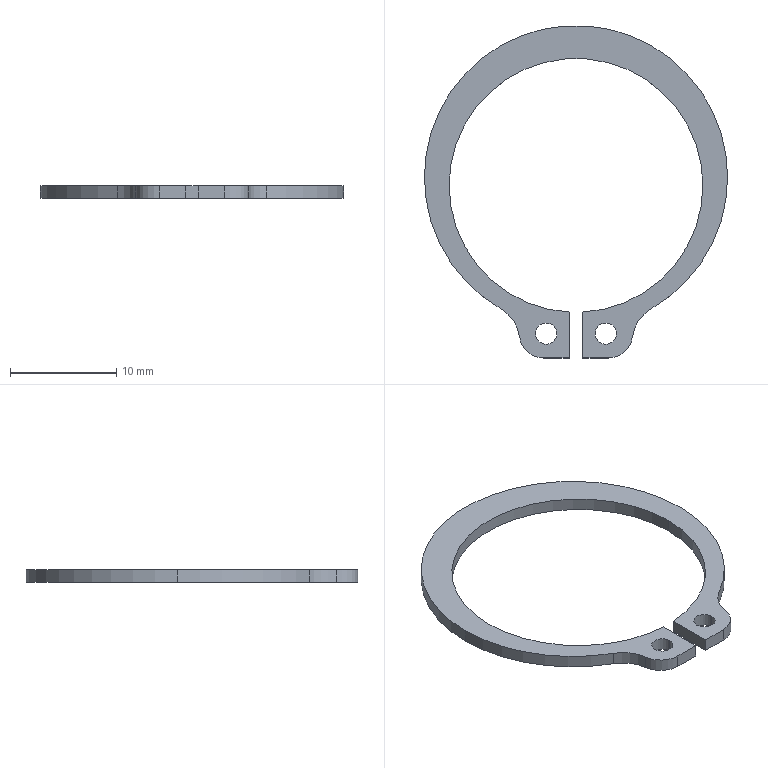Component | SolidWorks | RetainingRing25-1 | 1 solid | 20 faces | box 28.55 x 31.3 x 1.2 mm | volume 254 mm3 | cylinder 14 | plane 6 | commonest cylinder face diameters 2 x4 28.55 x3 23.9 x3 6.9 x2 4.6 x2
STEP:
#1=COLOUR_RGB('',0.7922,0.8196,0.9333);
#2=FILL_AREA_STYLE_COLOUR('',#1);
#3=FILL_AREA_STYLE('',(#2));
#4=SURFACE_STYLE_FILL_AREA(#3);
#5=SURFACE_SIDE_STYLE('',(#4));
#6=SURFACE_STYLE_USAGE(.BOTH.,#5);
#7=PRESENTATION_STYLE_ASSIGNMENT((#6));
#8=CARTESIAN_POINT('',(0.1607,-0.4136,-67.035));
#9=VERTEX_POINT('',#8);
#10=CARTESIAN_POINT('',(0.08192,-0.4136,-67.035));
#11=VERTEX_POINT('',#10);
#12=CARTESIAN_POINT('',(0.1213,-0.4136,-67.035));
#13=DIRECTION('',(0.,0.,-1.));
#14=DIRECTION('',(1.,0.,0.));
#15=AXIS2_PLACEMENT_3D('',#12,#13,#14);
#16=CIRCLE('',#15,0.03937);
#17=EDGE_CURVE('',#9,#11,#16,.T.);
#18=ORIENTED_EDGE('',*,*,#17,.T.);
#19=CARTESIAN_POINT('',(0.08192,-0.4136,-66.988));
#20=VERTEX_POINT('',#19);
#21=CARTESIAN_POINT('',(0.08192,-0.4136,-66.988));
#22=DIRECTION('',(0.,0.,1.));
#23=VECTOR('',#22,39.37);
#24=LINE('',#21,#23);
#25=EDGE_CURVE('',#11,#20,#24,.T.);
#26=ORIENTED_EDGE('',*,*,#25,.T.);
#27=CARTESIAN_POINT('',(0.1607,-0.4136,-66.988));
#28=VERTEX_POINT('',#27);
#29=CARTESIAN_POINT('',(0.1213,-0.4136,-66.988));
#30=DIRECTION('',(0.,0.,-1.));
#31=DIRECTION('',(1.,0.,0.));
#32=AXIS2_PLACEMENT_3D('',#29,#30,#31);
#33=CIRCLE('',#32,0.03937);
#34=EDGE_CURVE('',#28,#20,#33,.T.);
#35=ORIENTED_EDGE('',*,*,#34,.F.);
#36=CARTESIAN_POINT('',(0.1607,-0.4136,-66.988));
#37=DIRECTION('',(0.,0.,1.));
#38=VECTOR('',#37,39.37);
#39=LINE('',#36,#38);
#40=EDGE_CURVE('',#9,#28,#39,.T.);
#41=ORIENTED_EDGE('',*,*,#40,.F.);
#42=EDGE_LOOP('',(#18,#26,#35,#41));
#43=FACE_OUTER_BOUND('',#42,.T.);
#44=CARTESIAN_POINT('',(0.1213,-0.4136,-66.988));
#45=DIRECTION('',(0.,0.,1.));
#46=DIRECTION('',(1.,0.,0.));
#47=AXIS2_PLACEMENT_3D('',#44,#45,#46);
#48=CYLINDRICAL_SURFACE('',#47,0.03937);
#49=ADVANCED_FACE('',(#43),#48,.F.);
#50=CARTESIAN_POINT('',(0.3811,-0.4136,-67.035));
#51=VERTEX_POINT('',#50);
#52=CARTESIAN_POINT('',(0.3024,-0.4136,-67.035));
#53=VERTEX_POINT('',#52);
#54=CARTESIAN_POINT('',(0.3418,-0.4136,-67.035));
#55=DIRECTION('',(0.,0.,-1.));
#56=DIRECTION('',(1.,0.,0.));
#57=AXIS2_PLACEMENT_3D('',#54,#55,#56);
#58=CIRCLE('',#57,0.03937);
#59=EDGE_CURVE('',#51,#53,#58,.T.);
#60=ORIENTED_EDGE('',*,*,#59,.T.);
#61=CARTESIAN_POINT('',(0.3024,-0.4136,-66.988));
#62=VERTEX_POINT('',#61);
#63=CARTESIAN_POINT('',(0.3024,-0.4136,-66.988));
#64=DIRECTION('',(0.,0.,1.));
#65=VECTOR('',#64,39.37);
#66=LINE('',#63,#65);
#67=EDGE_CURVE('',#53,#62,#66,.T.);
#68=ORIENTED_EDGE('',*,*,#67,.T.);
#69=CARTESIAN_POINT('',(0.3811,-0.4136,-66.988));
#70=VERTEX_POINT('',#69);
#71=CARTESIAN_POINT('',(0.3418,-0.4136,-66.988));
#72=DIRECTION('',(0.,0.,-1.));
#73=DIRECTION('',(1.,0.,0.));
#74=AXIS2_PLACEMENT_3D('',#71,#72,#73);
#75=CIRCLE('',#74,0.03937);
#76=EDGE_CURVE('',#70,#62,#75,.T.);
#77=ORIENTED_EDGE('',*,*,#76,.F.);
#78=CARTESIAN_POINT('',(0.3811,-0.4136,-66.988));
#79=DIRECTION('',(0.,0.,1.));
#80=VECTOR('',#79,39.37);
#81=LINE('',#78,#80);
#82=EDGE_CURVE('',#51,#70,#81,.T.);
#83=ORIENTED_EDGE('',*,*,#82,.F.);
#84=EDGE_LOOP('',(#60,#68,#77,#83));
#85=FACE_OUTER_BOUND('',#84,.T.);
#86=CARTESIAN_POINT('',(0.3418,-0.4136,-66.988));
#87=DIRECTION('',(0.,0.,1.));
#88=DIRECTION('',(1.,0.,0.));
#89=AXIS2_PLACEMENT_3D('',#86,#87,#88);
#90=CYLINDRICAL_SURFACE('',#89,0.03937);
#91=ADVANCED_FACE('',(#85),#90,.F.);
#92=CARTESIAN_POINT('',(0.7935,0.1661,-67.035));
#93=VERTEX_POINT('',#92);
#94=CARTESIAN_POINT('',(-0.3305,0.1661,-67.035));
#95=VERTEX_POINT('',#94);
#96=CARTESIAN_POINT('',(0.2315,0.1661,-67.035));
#97=DIRECTION('',(0.,0.,1.));
#98=DIRECTION('',(1.,0.,0.));
#99=AXIS2_PLACEMENT_3D('',#96,#97,#98);
#100=CIRCLE('',#99,0.562);
#101=EDGE_CURVE('',#93,#95,#100,.T.);
#102=ORIENTED_EDGE('',*,*,#101,.T.);
#103=CARTESIAN_POINT('',(-0.3305,0.1661,-66.988));
#104=VERTEX_POINT('',#103);
#105=CARTESIAN_POINT('',(-0.3305,0.1661,-66.988));
#106=DIRECTION('',(0.,0.,1.));
#107=VECTOR('',#106,39.37);
#108=LINE('',#105,#107);
#109=EDGE_CURVE('',#95,#104,#108,.T.);
#110=ORIENTED_EDGE('',*,*,#109,.T.);
#111=CARTESIAN_POINT('',(0.7935,0.1661,-66.988));
#112=VERTEX_POINT('',#111);
#113=CARTESIAN_POINT('',(0.2315,0.1661,-66.988));
#114=DIRECTION('',(0.,0.,-1.));
#115=DIRECTION('',(1.,0.,0.));
#116=AXIS2_PLACEMENT_3D('',#113,#114,#115);
#117=CIRCLE('',#116,0.562);
#118=EDGE_CURVE('',#104,#112,#117,.T.);
#119=ORIENTED_EDGE('',*,*,#118,.T.);
#120=CARTESIAN_POINT('',(0.7935,0.1661,-66.988));
#121=DIRECTION('',(0.,0.,1.));
#122=VECTOR('',#121,39.37);
#123=LINE('',#120,#122);
#124=EDGE_CURVE('',#93,#112,#123,.T.);
#125=ORIENTED_EDGE('',*,*,#124,.F.);
#126=EDGE_LOOP('',(#102,#110,#119,#125));
#127=FACE_OUTER_BOUND('',#126,.T.);
#128=CARTESIAN_POINT('',(0.2315,0.1661,-66.988));
#129=DIRECTION('',(0.,0.,1.));
#130=DIRECTION('',(1.,0.,0.));
#131=AXIS2_PLACEMENT_3D('',#128,#129,#130);
#132=CYLINDRICAL_SURFACE('',#131,0.562);
#133=ADVANCED_FACE('',(#127),#132,.T.);
#134=CARTESIAN_POINT('',(0.509,-0.3226,-67.035));
#135=VERTEX_POINT('',#134);
#136=CARTESIAN_POINT('',(0.2315,0.1661,-67.035));
#137=DIRECTION('',(0.,0.,1.));
#138=DIRECTION('',(1.,0.,0.));
#139=AXIS2_PLACEMENT_3D('',#136,#137,#138);
#140=CIRCLE('',#139,0.562);
#141=EDGE_CURVE('',#135,#93,#140,.T.);
#142=ORIENTED_EDGE('',*,*,#141,.T.);
#143=ORIENTED_EDGE('',*,*,#124,.T.);
#144=CARTESIAN_POINT('',(0.509,-0.3226,-66.988));
#145=VERTEX_POINT('',#144);
#146=CARTESIAN_POINT('',(0.2315,0.1661,-66.988));
#147=DIRECTION('',(0.,0.,-1.));
#148=DIRECTION('',(1.,0.,0.));
#149=AXIS2_PLACEMENT_3D('',#146,#147,#148);
#150=CIRCLE('',#149,0.562);
#151=EDGE_CURVE('',#112,#145,#150,.T.);
#152=ORIENTED_EDGE('',*,*,#151,.T.);
#153=CARTESIAN_POINT('',(0.509,-0.3226,-66.988));
#154=DIRECTION('',(0.,0.,-1.));
#155=VECTOR('',#154,39.37);
#156=LINE('',#153,#155);
#157=EDGE_CURVE('',#145,#135,#156,.T.);
#158=ORIENTED_EDGE('',*,*,#157,.T.);
#159=EDGE_LOOP('',(#142,#143,#152,#158));
#160=FACE_OUTER_BOUND('',#159,.T.);
#161=CARTESIAN_POINT('',(0.2315,0.1661,-66.988));
#162=DIRECTION('',(0.,0.,1.));
#163=DIRECTION('',(1.,0.,0.));
#164=AXIS2_PLACEMENT_3D('',#161,#162,#163);
#165=CYLINDRICAL_SURFACE('',#164,0.562);
#166=ADVANCED_FACE('',(#160),#165,.T.);
#167=CARTESIAN_POINT('',(0.2059,-0.3342,-67.035));
#168=VERTEX_POINT('',#167);
#169=CARTESIAN_POINT('',(-0.2389,0.1356,-67.035));
#170=VERTEX_POINT('',#169);
#171=CARTESIAN_POINT('',(0.2315,0.1356,-67.035));
#172=DIRECTION('',(0.,0.,-1.));
#173=DIRECTION('',(1.,0.,0.));
#174=AXIS2_PLACEMENT_3D('',#171,#172,#173);
#175=CIRCLE('',#174,0.4705);
#176=EDGE_CURVE('',#168,#170,#175,.T.);
#177=ORIENTED_EDGE('',*,*,#176,.T.);
#178=CARTESIAN_POINT('',(-0.2389,0.1356,-66.988));
#179=VERTEX_POINT('',#178);
#180=CARTESIAN_POINT('',(-0.2389,0.1356,-66.988));
#181=DIRECTION('',(0.,0.,1.));
#182=VECTOR('',#181,39.37);
#183=LINE('',#180,#182);
#184=EDGE_CURVE('',#170,#179,#183,.T.);
#185=ORIENTED_EDGE('',*,*,#184,.T.);
#186=CARTESIAN_POINT('',(0.2059,-0.3342,-66.988));
#187=VERTEX_POINT('',#186);
#188=CARTESIAN_POINT('',(0.2315,0.1356,-66.988));
#189=DIRECTION('',(0.,0.,-1.));
#190=DIRECTION('',(1.,0.,0.));
#191=AXIS2_PLACEMENT_3D('',#188,#189,#190);
#192=CIRCLE('',#191,0.4705);
#193=EDGE_CURVE('',#187,#179,#192,.T.);
#194=ORIENTED_EDGE('',*,*,#193,.F.);
#195=CARTESIAN_POINT('',(0.2059,-0.3342,-66.988));
#196=DIRECTION('',(0.,0.,1.));
#197=VECTOR('',#196,39.37);
#198=LINE('',#195,#197);
#199=EDGE_CURVE('',#168,#187,#198,.T.);
#200=ORIENTED_EDGE('',*,*,#199,.F.);
#201=EDGE_LOOP('',(#177,#185,#194,#200));
#202=FACE_OUTER_BOUND('',#201,.T.);
#203=CARTESIAN_POINT('',(0.2315,0.1356,-66.988));
#204=DIRECTION('',(0.,0.,1.));
#205=DIRECTION('',(1.,0.,0.));
#206=AXIS2_PLACEMENT_3D('',#203,#204,#205);
#207=CYLINDRICAL_SURFACE('',#206,0.4705);
#208=ADVANCED_FACE('',(#202),#207,.F.);
#209=ORIENTED_EDGE('',*,*,#184,.F.);
#210=CARTESIAN_POINT('',(0.702,0.1356,-67.035));
#211=VERTEX_POINT('',#210);
#212=CARTESIAN_POINT('',(0.2315,0.1356,-67.035));
#213=DIRECTION('',(0.,0.,-1.));
#214=DIRECTION('',(1.,0.,0.));
#215=AXIS2_PLACEMENT_3D('',#212,#213,#214);
#216=CIRCLE('',#215,0.4705);
#217=EDGE_CURVE('',#170,#211,#216,.T.);
#218=ORIENTED_EDGE('',*,*,#217,.T.);
#219=CARTESIAN_POINT('',(0.702,0.1356,-66.988));
#220=VERTEX_POINT('',#219);
#221=CARTESIAN_POINT('',(0.702,0.1356,-66.988));
#222=DIRECTION('',(0.,0.,1.));
#223=VECTOR('',#222,39.37);
#224=LINE('',#221,#223);
#225=EDGE_CURVE('',#211,#220,#224,.T.);
#226=ORIENTED_EDGE('',*,*,#225,.T.);
#227=CARTESIAN_POINT('',(0.2315,0.1356,-66.988));
#228=DIRECTION('',(0.,0.,-1.));
#229=DIRECTION('',(1.,0.,0.));
#230=AXIS2_PLACEMENT_3D('',#227,#228,#229);
#231=CIRCLE('',#230,0.4705);
#232=EDGE_CURVE('',#179,#220,#231,.T.);
#233=ORIENTED_EDGE('',*,*,#232,.F.);
#234=EDGE_LOOP('',(#209,#218,#226,#233));
#235=FACE_OUTER_BOUND('',#234,.T.);
#236=CARTESIAN_POINT('',(0.2315,0.1356,-66.988));
#237=DIRECTION('',(0.,0.,1.));
#238=DIRECTION('',(1.,0.,0.));
#239=AXIS2_PLACEMENT_3D('',#236,#237,#238);
#240=CYLINDRICAL_SURFACE('',#239,0.4705);
#241=ADVANCED_FACE('',(#235),#240,.F.);
#242=ORIENTED_EDGE('',*,*,#17,.F.);
#243=CARTESIAN_POINT('',(0.1213,-0.4136,-67.035));
#244=DIRECTION('',(0.,0.,-1.));
#245=DIRECTION('',(1.,0.,0.));
#246=AXIS2_PLACEMENT_3D('',#243,#244,#245);
#247=CIRCLE('',#246,0.03937);
#248=EDGE_CURVE('',#11,#9,#247,.T.);
#249=ORIENTED_EDGE('',*,*,#248,.F.);
#250=EDGE_LOOP('',(#242,#249));
#251=FACE_BOUND('',#250,.T.);
#252=ORIENTED_EDGE('',*,*,#59,.F.);
#253=CARTESIAN_POINT('',(0.3418,-0.4136,-67.035));
#254=DIRECTION('',(0.,0.,-1.));
#255=DIRECTION('',(1.,0.,0.));
#256=AXIS2_PLACEMENT_3D('',#253,#254,#255);
#257=CIRCLE('',#256,0.03937);
#258=EDGE_CURVE('',#53,#51,#257,.T.);
#259=ORIENTED_EDGE('',*,*,#258,.F.);
#260=EDGE_LOOP('',(#252,#259));
#261=FACE_BOUND('',#260,.T.);
#262=CARTESIAN_POINT('',(-0.04591,-0.3226,-67.035));
#263=VERTEX_POINT('',#262);
#264=CARTESIAN_POINT('',(0.02188,-0.4245,-67.035));
#265=VERTEX_POINT('',#264);
#266=CARTESIAN_POINT('',(-0.113,-0.4408,-67.035));
#267=DIRECTION('',(0.,0.,-1.));
#268=DIRECTION('',(1.,-0.,0.));
#269=AXIS2_PLACEMENT_3D('',#266,#267,#268);
#270=CIRCLE('',#269,0.1358);
#271=EDGE_CURVE('',#263,#265,#270,.T.);
#272=ORIENTED_EDGE('',*,*,#271,.F.);
#273=CARTESIAN_POINT('',(0.2315,0.1661,-67.035));
#274=DIRECTION('',(0.,0.,1.));
#275=DIRECTION('',(1.,0.,0.));
#276=AXIS2_PLACEMENT_3D('',#273,#274,#275);
#277=CIRCLE('',#276,0.562);
#278=EDGE_CURVE('',#95,#263,#277,.T.);
#279=ORIENTED_EDGE('',*,*,#278,.F.);
#280=ORIENTED_EDGE('',*,*,#101,.F.);
#281=ORIENTED_EDGE('',*,*,#141,.F.);
#282=CARTESIAN_POINT('',(0.4412,-0.4245,-67.035));
#283=VERTEX_POINT('',#282);
#284=CARTESIAN_POINT('',(0.576,-0.4408,-67.035));
#285=DIRECTION('',(0.,0.,-1.));
#286=DIRECTION('',(1.,-0.,0.));
#287=AXIS2_PLACEMENT_3D('',#284,#285,#286);
#288=CIRCLE('',#287,0.1358);
#289=EDGE_CURVE('',#283,#135,#288,.T.);
#290=ORIENTED_EDGE('',*,*,#289,.F.);
#291=CARTESIAN_POINT('',(0.3513,-0.5042,-67.035));
#292=VERTEX_POINT('',#291);
#293=CARTESIAN_POINT('',(0.3513,-0.4136,-67.035));
#294=DIRECTION('',(0.,0.,1.));
#295=DIRECTION('',(1.,0.,0.));
#296=AXIS2_PLACEMENT_3D('',#293,#294,#295);
#297=CIRCLE('',#296,0.09055);
#298=EDGE_CURVE('',#292,#283,#297,.T.);
#299=ORIENTED_EDGE('',*,*,#298,.F.);
#300=CARTESIAN_POINT('',(0.2571,-0.5042,-67.035));
#301=VERTEX_POINT('',#300);
#302=CARTESIAN_POINT('',(0.2315,-0.5042,-67.035));
#303=DIRECTION('',(1.,0.,0.));
#304=VECTOR('',#303,39.37);
#305=LINE('',#302,#304);
#306=EDGE_CURVE('',#301,#292,#305,.T.);
#307=ORIENTED_EDGE('',*,*,#306,.F.);
#308=CARTESIAN_POINT('',(0.2571,-0.3342,-67.035));
#309=VERTEX_POINT('',#308);
#310=CARTESIAN_POINT('',(0.2571,0.1356,-67.035));
#311=DIRECTION('',(0.,-1.,0.));
#312=VECTOR('',#311,39.37);
#313=LINE('',#310,#312);
#314=EDGE_CURVE('',#309,#301,#313,.T.);
#315=ORIENTED_EDGE('',*,*,#314,.F.);
#316=CARTESIAN_POINT('',(0.2315,0.1356,-67.035));
#317=DIRECTION('',(0.,0.,-1.));
#318=DIRECTION('',(1.,0.,0.));
#319=AXIS2_PLACEMENT_3D('',#316,#317,#318);
#320=CIRCLE('',#319,0.4705);
#321=EDGE_CURVE('',#211,#309,#320,.T.);
#322=ORIENTED_EDGE('',*,*,#321,.F.);
#323=ORIENTED_EDGE('',*,*,#217,.F.);
#324=ORIENTED_EDGE('',*,*,#176,.F.);
#325=CARTESIAN_POINT('',(0.2059,-0.5042,-67.035));
#326=VERTEX_POINT('',#325);
#327=CARTESIAN_POINT('',(0.2059,0.1356,-67.035));
#328=DIRECTION('',(0.,1.,0.));
#329=VECTOR('',#328,39.37);
#330=LINE('',#327,#329);
#331=EDGE_CURVE('',#326,#168,#330,.T.);
#332=ORIENTED_EDGE('',*,*,#331,.F.);
#333=CARTESIAN_POINT('',(0.1118,-0.5042,-67.035));
#334=VERTEX_POINT('',#333);
#335=CARTESIAN_POINT('',(0.2315,-0.5042,-67.035));
#336=DIRECTION('',(1.,0.,0.));
#337=VECTOR('',#336,39.37);
#338=LINE('',#335,#337);
#339=EDGE_CURVE('',#334,#326,#338,.T.);
#340=ORIENTED_EDGE('',*,*,#339,.F.);
#341=CARTESIAN_POINT('',(0.1118,-0.4136,-67.035));
#342=DIRECTION('',(0.,0.,1.));
#343=DIRECTION('',(1.,0.,0.));
#344=AXIS2_PLACEMENT_3D('',#341,#342,#343);
#345=CIRCLE('',#344,0.09055);
#346=EDGE_CURVE('',#265,#334,#345,.T.);
#347=ORIENTED_EDGE('',*,*,#346,.F.);
#348=EDGE_LOOP('',(#272,#279,#280,#281,#290,#299,#307,#315,#322,#323,#324,#332,#340,#347));
#349=FACE_OUTER_BOUND('',#348,.T.);
#350=CARTESIAN_POINT('',(0.2315,0.1356,-67.035));
#351=DIRECTION('',(0.,0.,1.));
#352=DIRECTION('',(1.,0.,0.));
#353=AXIS2_PLACEMENT_3D('',#350,#351,#352);
#354=PLANE('',#353);
#355=ADVANCED_FACE('',(#251,#261,#349),#354,.F.);
#356=ORIENTED_EDGE('',*,*,#25,.F.);
#357=ORIENTED_EDGE('',*,*,#248,.T.);
#358=ORIENTED_EDGE('',*,*,#40,.T.);
#359=CARTESIAN_POINT('',(0.1213,-0.4136,-66.988));
#360=DIRECTION('',(0.,0.,-1.));
#361=DIRECTION('',(1.,0.,0.));
#362=AXIS2_PLACEMENT_3D('',#359,#360,#361);
#363=CIRCLE('',#362,0.03937);
#364=EDGE_CURVE('',#20,#28,#363,.T.);
#365=ORIENTED_EDGE('',*,*,#364,.F.);
#366=EDGE_LOOP('',(#356,#357,#358,#365));
#367=FACE_OUTER_BOUND('',#366,.T.);
#368=CARTESIAN_POINT('',(0.1213,-0.4136,-66.988));
#369=DIRECTION('',(0.,0.,1.));
#370=DIRECTION('',(1.,0.,0.));
#371=AXIS2_PLACEMENT_3D('',#368,#369,#370);
#372=CYLINDRICAL_SURFACE('',#371,0.03937);
#373=ADVANCED_FACE('',(#367),#372,.F.);
#374=ORIENTED_EDGE('',*,*,#67,.F.);
#375=ORIENTED_EDGE('',*,*,#258,.T.);
#376=ORIENTED_EDGE('',*,*,#82,.T.);
#377=CARTESIAN_POINT('',(0.3418,-0.4136,-66.988));
#378=DIRECTION('',(0.,0.,-1.));
#379=DIRECTION('',(1.,0.,0.));
#380=AXIS2_PLACEMENT_3D('',#377,#378,#379);
#381=CIRCLE('',#380,0.03937);
#382=EDGE_CURVE('',#62,#70,#381,.T.);
#383=ORIENTED_EDGE('',*,*,#382,.F.);
#384=EDGE_LOOP('',(#374,#375,#376,#383));
#385=FACE_OUTER_BOUND('',#384,.T.);
#386=CARTESIAN_POINT('',(0.3418,-0.4136,-66.988));
#387=DIRECTION('',(0.,0.,1.));
#388=DIRECTION('',(1.,0.,0.));
#389=AXIS2_PLACEMENT_3D('',#386,#387,#388);
#390=CYLINDRICAL_SURFACE('',#389,0.03937);
#391=ADVANCED_FACE('',(#385),#390,.F.);
#392=CARTESIAN_POINT('',(0.02188,-0.4245,-66.988));
#393=VERTEX_POINT('',#392);
#394=CARTESIAN_POINT('',(0.02188,-0.4245,-66.988));
#395=DIRECTION('',(0.,0.,-1.));
#396=VECTOR('',#395,39.37);
#397=LINE('',#394,#396);
#398=EDGE_CURVE('',#393,#265,#397,.T.);
#399=ORIENTED_EDGE('',*,*,#398,.F.);
#400=CARTESIAN_POINT('',(-0.04591,-0.3226,-66.988));
#401=VERTEX_POINT('',#400);
#402=CARTESIAN_POINT('',(-0.113,-0.4408,-66.988));
#403=DIRECTION('',(0.,0.,-1.));
#404=DIRECTION('',(1.,-0.,0.));
#405=AXIS2_PLACEMENT_3D('',#402,#403,#404);
#406=CIRCLE('',#405,0.1358);
#407=EDGE_CURVE('',#401,#393,#406,.T.);
#408=ORIENTED_EDGE('',*,*,#407,.F.);
#409=CARTESIAN_POINT('',(-0.04591,-0.3226,-66.988));
#410=DIRECTION('',(0.,0.,1.));
#411=VECTOR('',#410,39.37);
#412=LINE('',#409,#411);
#413=EDGE_CURVE('',#263,#401,#412,.T.);
#414=ORIENTED_EDGE('',*,*,#413,.F.);
#415=ORIENTED_EDGE('',*,*,#271,.T.);
#416=EDGE_LOOP('',(#399,#408,#414,#415));
#417=FACE_OUTER_BOUND('',#416,.T.);
#418=CARTESIAN_POINT('',(-0.113,-0.4408,-66.988));
#419=DIRECTION('',(0.,0.,1.));
#420=DIRECTION('',(1.,0.,0.));
#421=AXIS2_PLACEMENT_3D('',#418,#419,#420);
#422=CYLINDRICAL_SURFACE('',#421,0.1358);
#423=ADVANCED_FACE('',(#417),#422,.F.);
#424=ORIENTED_EDGE('',*,*,#109,.F.);
#425=ORIENTED_EDGE('',*,*,#278,.T.);
#426=ORIENTED_EDGE('',*,*,#413,.T.);
#427=CARTESIAN_POINT('',(0.2315,0.1661,-66.988));
#428=DIRECTION('',(0.,0.,-1.));
#429=DIRECTION('',(1.,0.,0.));
#430=AXIS2_PLACEMENT_3D('',#427,#428,#429);
#431=CIRCLE('',#430,0.562);
#432=EDGE_CURVE('',#401,#104,#431,.T.);
#433=ORIENTED_EDGE('',*,*,#432,.T.);
#434=EDGE_LOOP('',(#424,#425,#426,#433));
#435=FACE_OUTER_BOUND('',#434,.T.);
#436=CARTESIAN_POINT('',(0.2315,0.1661,-66.988));
#437=DIRECTION('',(0.,0.,1.));
#438=DIRECTION('',(1.,0.,0.));
#439=AXIS2_PLACEMENT_3D('',#436,#437,#438);
#440=CYLINDRICAL_SURFACE('',#439,0.562);
#441=ADVANCED_FACE('',(#435),#440,.T.);
#442=ORIENTED_EDGE('',*,*,#157,.F.);
#443=CARTESIAN_POINT('',(0.4412,-0.4245,-66.988));
#444=VERTEX_POINT('',#443);
#445=CARTESIAN_POINT('',(0.576,-0.4408,-66.988));
#446=DIRECTION('',(0.,0.,-1.));
#447=DIRECTION('',(1.,-0.,0.));
#448=AXIS2_PLACEMENT_3D('',#445,#446,#447);
#449=CIRCLE('',#448,0.1358);
#450=EDGE_CURVE('',#444,#145,#449,.T.);
#451=ORIENTED_EDGE('',*,*,#450,.F.);
#452=CARTESIAN_POINT('',(0.4412,-0.4245,-66.988));
#453=DIRECTION('',(0.,0.,1.));
#454=VECTOR('',#453,39.37);
#455=LINE('',#452,#454);
#456=EDGE_CURVE('',#283,#444,#455,.T.);
#457=ORIENTED_EDGE('',*,*,#456,.F.);
#458=ORIENTED_EDGE('',*,*,#289,.T.);
#459=EDGE_LOOP('',(#442,#451,#457,#458));
#460=FACE_OUTER_BOUND('',#459,.T.);
#461=CARTESIAN_POINT('',(0.576,-0.4408,-66.988));
#462=DIRECTION('',(0.,0.,1.));
#463=DIRECTION('',(1.,0.,0.));
#464=AXIS2_PLACEMENT_3D('',#461,#462,#463);
#465=CYLINDRICAL_SURFACE('',#464,0.1358);
#466=ADVANCED_FACE('',(#460),#465,.F.);
#467=CARTESIAN_POINT('',(0.3513,-0.5042,-66.988));
#468=VERTEX_POINT('',#467);
#469=CARTESIAN_POINT('',(0.3513,-0.4136,-66.988));
#470=DIRECTION('',(0.,0.,-1.));
#471=DIRECTION('',(1.,0.,0.));
#472=AXIS2_PLACEMENT_3D('',#469,#470,#471);
#473=CIRCLE('',#472,0.09055);
#474=EDGE_CURVE('',#444,#468,#473,.T.);
#475=ORIENTED_EDGE('',*,*,#474,.T.);
#476=CARTESIAN_POINT('',(0.3513,-0.5042,-66.988));
#477=DIRECTION('',(0.,0.,-1.));
#478=VECTOR('',#477,39.37);
#479=LINE('',#476,#478);
#480=EDGE_CURVE('',#468,#292,#479,.T.);
#481=ORIENTED_EDGE('',*,*,#480,.T.);
#482=ORIENTED_EDGE('',*,*,#298,.T.);
#483=ORIENTED_EDGE('',*,*,#456,.T.);
#484=EDGE_LOOP('',(#475,#481,#482,#483));
#485=FACE_OUTER_BOUND('',#484,.T.);
#486=CARTESIAN_POINT('',(0.3513,-0.4136,-66.988));
#487=DIRECTION('',(0.,0.,1.));
#488=DIRECTION('',(1.,0.,0.));
#489=AXIS2_PLACEMENT_3D('',#486,#487,#488);
#490=CYLINDRICAL_SURFACE('',#489,0.09055);
#491=ADVANCED_FACE('',(#485),#490,.T.);
#492=CARTESIAN_POINT('',(0.2571,-0.5042,-66.988));
#493=VERTEX_POINT('',#492);
#494=CARTESIAN_POINT('',(0.2571,-0.5042,-66.988));
#495=DIRECTION('',(-1.,0.,0.));
#496=VECTOR('',#495,39.37);
#497=LINE('',#494,#496);
#498=EDGE_CURVE('',#468,#493,#497,.T.);
#499=ORIENTED_EDGE('',*,*,#498,.T.);
#500=CARTESIAN_POINT('',(0.2571,-0.5042,-66.988));
#501=DIRECTION('',(0.,0.,-1.));
#502=VECTOR('',#501,39.37);
#503=LINE('',#500,#502);
#504=EDGE_CURVE('',#493,#301,#503,.T.);
#505=ORIENTED_EDGE('',*,*,#504,.T.);
#506=ORIENTED_EDGE('',*,*,#306,.T.);
#507=ORIENTED_EDGE('',*,*,#480,.F.);
#508=EDGE_LOOP('',(#499,#505,#506,#507));
#509=FACE_OUTER_BOUND('',#508,.T.);
#510=CARTESIAN_POINT('',(0.2571,-0.5042,-66.988));
#511=DIRECTION('',(0.,-1.,0.));
#512=DIRECTION('',(1.,0.,0.));
#513=AXIS2_PLACEMENT_3D('',#510,#511,#512);
#514=PLANE('',#513);
#515=ADVANCED_FACE('',(#509),#514,.T.);
#516=CARTESIAN_POINT('',(0.2571,-0.3342,-66.988));
#517=VERTEX_POINT('',#516);
#518=CARTESIAN_POINT('',(0.2571,-0.3342,-66.988));
#519=DIRECTION('',(0.,1.,0.));
#520=VECTOR('',#519,39.37);
#521=LINE('',#518,#520);
#522=EDGE_CURVE('',#493,#517,#521,.T.);
#523=ORIENTED_EDGE('',*,*,#522,.T.);
#524=CARTESIAN_POINT('',(0.2571,-0.3342,-66.988));
#525=DIRECTION('',(0.,0.,-1.));
#526=VECTOR('',#525,39.37);
#527=LINE('',#524,#526);
#528=EDGE_CURVE('',#517,#309,#527,.T.);
#529=ORIENTED_EDGE('',*,*,#528,.T.);
#530=ORIENTED_EDGE('',*,*,#314,.T.);
#531=ORIENTED_EDGE('',*,*,#504,.F.);
#532=EDGE_LOOP('',(#523,#529,#530,#531));
#533=FACE_OUTER_BOUND('',#532,.T.);
#534=CARTESIAN_POINT('',(0.2571,-0.3342,-66.988));
#535=DIRECTION('',(-1.,0.,0.));
#536=DIRECTION('',(0.,0.,1.));
#537=AXIS2_PLACEMENT_3D('',#534,#535,#536);
#538=PLANE('',#537);
#539=ADVANCED_FACE('',(#533),#538,.T.);
#540=ORIENTED_EDGE('',*,*,#225,.F.);
#541=ORIENTED_EDGE('',*,*,#321,.T.);
#542=ORIENTED_EDGE('',*,*,#528,.F.);
#543=CARTESIAN_POINT('',(0.2315,0.1356,-66.988));
#544=DIRECTION('',(0.,0.,-1.));
#545=DIRECTION('',(1.,0.,0.));
#546=AXIS2_PLACEMENT_3D('',#543,#544,#545);
#547=CIRCLE('',#546,0.4705);
#548=EDGE_CURVE('',#220,#517,#547,.T.);
#549=ORIENTED_EDGE('',*,*,#548,.F.);
#550=EDGE_LOOP('',(#540,#541,#542,#549));
#551=FACE_OUTER_BOUND('',#550,.T.);
#552=CARTESIAN_POINT('',(0.2315,0.1356,-66.988));
#553=DIRECTION('',(0.,0.,1.));
#554=DIRECTION('',(1.,0.,0.));
#555=AXIS2_PLACEMENT_3D('',#552,#553,#554);
#556=CYLINDRICAL_SURFACE('',#555,0.4705);
#557=ADVANCED_FACE('',(#551),#556,.F.);
#558=CARTESIAN_POINT('',(0.2059,-0.5042,-66.988));
#559=VERTEX_POINT('',#558);
#560=CARTESIAN_POINT('',(0.2059,-0.5042,-66.988));
#561=DIRECTION('',(0.,-1.,0.));
#562=VECTOR('',#561,39.37);
#563=LINE('',#560,#562);
#564=EDGE_CURVE('',#187,#559,#563,.T.);
#565=ORIENTED_EDGE('',*,*,#564,.T.);
#566=CARTESIAN_POINT('',(0.2059,-0.5042,-66.988));
#567=DIRECTION('',(0.,0.,-1.));
#568=VECTOR('',#567,39.37);
#569=LINE('',#566,#568);
#570=EDGE_CURVE('',#559,#326,#569,.T.);
#571=ORIENTED_EDGE('',*,*,#570,.T.);
#572=ORIENTED_EDGE('',*,*,#331,.T.);
#573=ORIENTED_EDGE('',*,*,#199,.T.);
#574=EDGE_LOOP('',(#565,#571,#572,#573));
#575=FACE_OUTER_BOUND('',#574,.T.);
#576=CARTESIAN_POINT('',(0.2059,-0.5042,-66.988));
#577=DIRECTION('',(1.,0.,0.));
#578=DIRECTION('',(-0.,1.,0.));
#579=AXIS2_PLACEMENT_3D('',#576,#577,#578);
#580=PLANE('',#579);
#581=ADVANCED_FACE('',(#575),#580,.T.);
#582=CARTESIAN_POINT('',(0.1118,-0.5042,-66.988));
#583=VERTEX_POINT('',#582);
#584=CARTESIAN_POINT('',(0.1118,-0.5042,-66.988));
#585=DIRECTION('',(-1.,0.,0.));
#586=VECTOR('',#585,39.37);
#587=LINE('',#584,#586);
#588=EDGE_CURVE('',#559,#583,#587,.T.);
#589=ORIENTED_EDGE('',*,*,#588,.T.);
#590=CARTESIAN_POINT('',(0.1118,-0.5042,-66.988));
#591=DIRECTION('',(0.,0.,-1.));
#592=VECTOR('',#591,39.37);
#593=LINE('',#590,#592);
#594=EDGE_CURVE('',#583,#334,#593,.T.);
#595=ORIENTED_EDGE('',*,*,#594,.T.);
#596=ORIENTED_EDGE('',*,*,#339,.T.);
#597=ORIENTED_EDGE('',*,*,#570,.F.);
#598=EDGE_LOOP('',(#589,#595,#596,#597));
#599=FACE_OUTER_BOUND('',#598,.T.);
#600=CARTESIAN_POINT('',(0.1118,-0.5042,-66.988));
#601=DIRECTION('',(0.,-1.,0.));
#602=DIRECTION('',(1.,0.,0.));
#603=AXIS2_PLACEMENT_3D('',#600,#601,#602);
#604=PLANE('',#603);
#605=ADVANCED_FACE('',(#599),#604,.T.);
#606=CARTESIAN_POINT('',(0.1118,-0.4136,-66.988));
#607=DIRECTION('',(0.,0.,-1.));
#608=DIRECTION('',(1.,0.,0.));
#609=AXIS2_PLACEMENT_3D('',#606,#607,#608);
#610=CIRCLE('',#609,0.09055);
#611=EDGE_CURVE('',#583,#393,#610,.T.);
#612=ORIENTED_EDGE('',*,*,#611,.T.);
#613=ORIENTED_EDGE('',*,*,#398,.T.);
#614=ORIENTED_EDGE('',*,*,#346,.T.);
#615=ORIENTED_EDGE('',*,*,#594,.F.);
#616=EDGE_LOOP('',(#612,#613,#614,#615));
#617=FACE_OUTER_BOUND('',#616,.T.);
#618=CARTESIAN_POINT('',(0.1118,-0.4136,-66.988));
#619=DIRECTION('',(0.,0.,1.));
#620=DIRECTION('',(1.,0.,0.));
#621=AXIS2_PLACEMENT_3D('',#618,#619,#620);
#622=CYLINDRICAL_SURFACE('',#621,0.09055);
#623=ADVANCED_FACE('',(#617),#622,.T.);
#624=ORIENTED_EDGE('',*,*,#34,.T.);
#625=ORIENTED_EDGE('',*,*,#364,.T.);
#626=EDGE_LOOP('',(#624,#625));
#627=FACE_BOUND('',#626,.T.);
#628=ORIENTED_EDGE('',*,*,#76,.T.);
#629=ORIENTED_EDGE('',*,*,#382,.T.);
#630=EDGE_LOOP('',(#628,#629));
#631=FACE_BOUND('',#630,.T.);
#632=ORIENTED_EDGE('',*,*,#474,.F.);
#633=ORIENTED_EDGE('',*,*,#450,.T.);
#634=ORIENTED_EDGE('',*,*,#151,.F.);
#635=ORIENTED_EDGE('',*,*,#118,.F.);
#636=ORIENTED_EDGE('',*,*,#432,.F.);
#637=ORIENTED_EDGE('',*,*,#407,.T.);
#638=ORIENTED_EDGE('',*,*,#611,.F.);
#639=ORIENTED_EDGE('',*,*,#588,.F.);
#640=ORIENTED_EDGE('',*,*,#564,.F.);
#641=ORIENTED_EDGE('',*,*,#193,.T.);
#642=ORIENTED_EDGE('',*,*,#232,.T.);
#643=ORIENTED_EDGE('',*,*,#548,.T.);
#644=ORIENTED_EDGE('',*,*,#522,.F.);
#645=ORIENTED_EDGE('',*,*,#498,.F.);
#646=EDGE_LOOP('',(#632,#633,#634,#635,#636,#637,#638,#639,#640,#641,#642,#643,#644,#645));
#647=FACE_OUTER_BOUND('',#646,.T.);
#648=CARTESIAN_POINT('',(0.2315,0.1356,-66.988));
#649=DIRECTION('',(0.,0.,1.));
#650=DIRECTION('',(1.,0.,0.));
#651=AXIS2_PLACEMENT_3D('',#648,#649,#650);
#652=PLANE('',#651);
#653=ADVANCED_FACE('',(#627,#631,#647),#652,.T.);
#654=CLOSED_SHELL('',(#49,#91,#133,#166,#208,#241,#355,#373,#391,#423,#441,#466,#491,#515,#539,#557,#581,#605,#623,#653));
#655=MANIFOLD_SOLID_BREP('',#654);
#656=STYLED_ITEM('',(#7),#655);
#657=(LENGTH_UNIT()NAMED_UNIT(*)SI_UNIT($,.METRE.));
#658=LENGTH_MEASURE_WITH_UNIT(LENGTH_MEASURE(0.0254),#657);
#659=DIMENSIONAL_EXPONENTS(1.,0.,0.,0.,0.,0.,0.);
#660=(CONVERSION_BASED_UNIT('',#658)LENGTH_UNIT()NAMED_UNIT(#659));
#661=UNCERTAINTY_MEASURE_WITH_UNIT(LENGTH_MEASURE(0.00001),#660,'','');
#662=(NAMED_UNIT(*)PLANE_ANGLE_UNIT()SI_UNIT($,.RADIAN.));
#663=(NAMED_UNIT(*)SI_UNIT($,.STERADIAN.)SOLID_ANGLE_UNIT());
#664=(GEOMETRIC_REPRESENTATION_CONTEXT(3)GLOBAL_UNCERTAINTY_ASSIGNED_CONTEXT((#661))GLOBAL_UNIT_ASSIGNED_CONTEXT((#660,#662,#663))REPRESENTATION_CONTEXT('',''));
#665=MECHANICAL_DESIGN_GEOMETRIC_PRESENTATION_REPRESENTATION('',(#656),#664);
#666=PRESENTATION_LAYER_ASSIGNMENT('','',(#656));
#667=CARTESIAN_POINT('',(0.,0.,0.));
#668=DIRECTION('',(0.,0.,1.));
#669=DIRECTION('',(1.,0.,0.));
#670=AXIS2_PLACEMENT_3D('',#667,#668,#669);
#671=(LENGTH_UNIT()NAMED_UNIT(*)SI_UNIT($,.METRE.));
#672=LENGTH_MEASURE_WITH_UNIT(LENGTH_MEASURE(0.0254),#671);
#673=DIMENSIONAL_EXPONENTS(1.,0.,0.,0.,0.,0.,0.);
#674=(CONVERSION_BASED_UNIT('',#672)LENGTH_UNIT()NAMED_UNIT(#673));
#675=UNCERTAINTY_MEASURE_WITH_UNIT(LENGTH_MEASURE(0.00001),#674,'','');
#676=(NAMED_UNIT(*)PLANE_ANGLE_UNIT()SI_UNIT($,.RADIAN.));
#677=(NAMED_UNIT(*)SI_UNIT($,.STERADIAN.)SOLID_ANGLE_UNIT());
#678=(GEOMETRIC_REPRESENTATION_CONTEXT(3)GLOBAL_UNCERTAINTY_ASSIGNED_CONTEXT((#675))GLOBAL_UNIT_ASSIGNED_CONTEXT((#674,#676,#677))REPRESENTATION_CONTEXT('',''));
#679=ADVANCED_BREP_SHAPE_REPRESENTATION('',(#655,#670),#678);